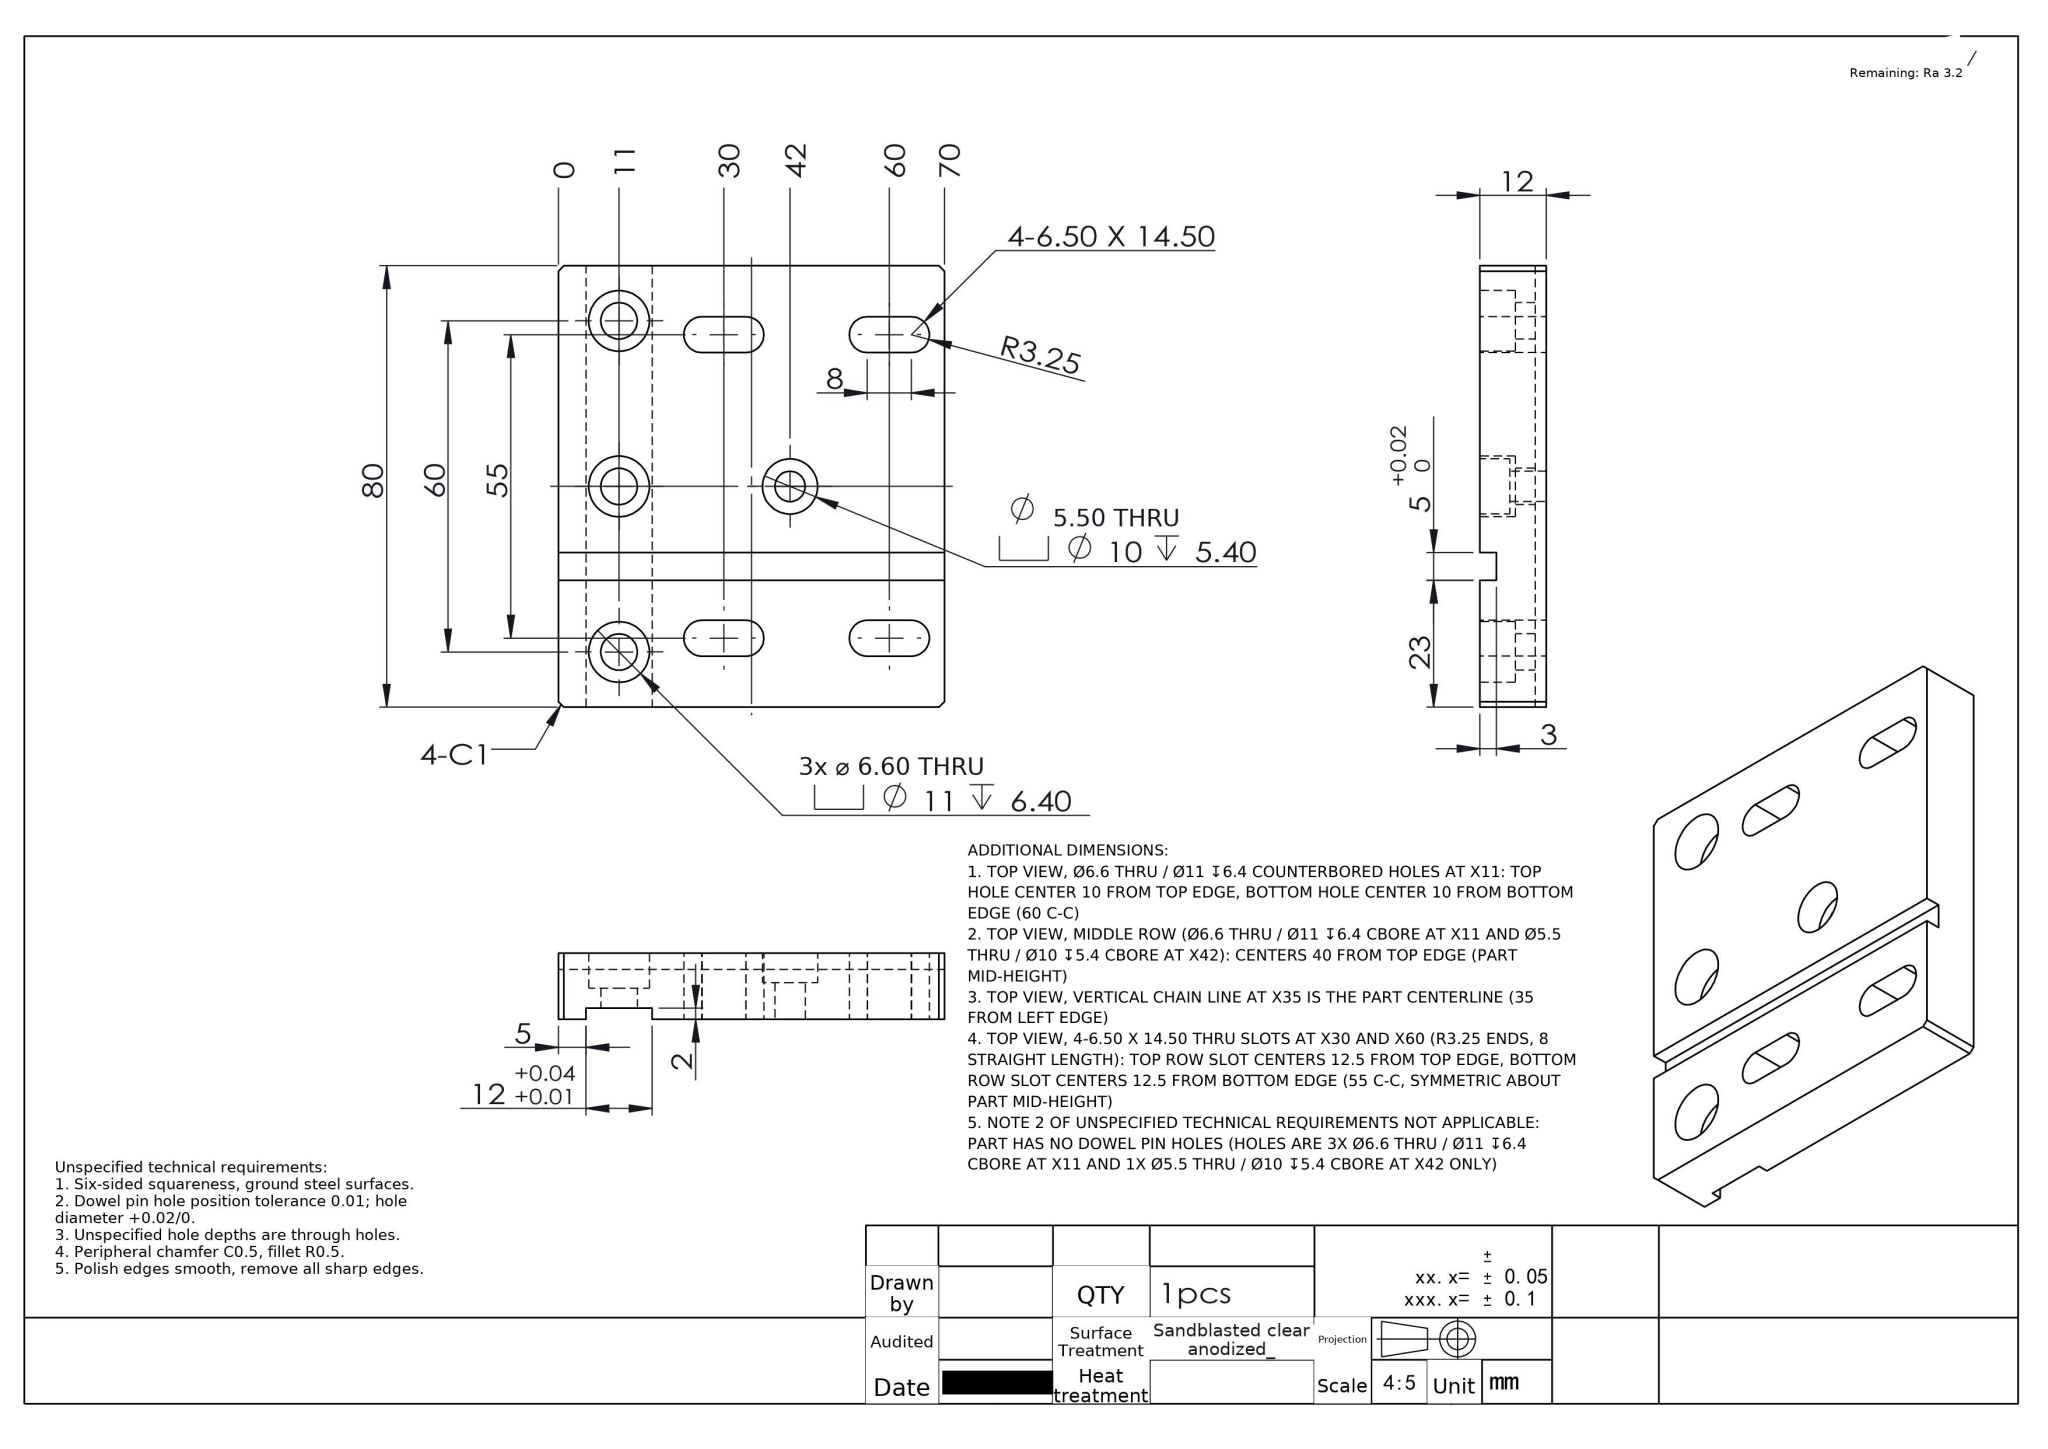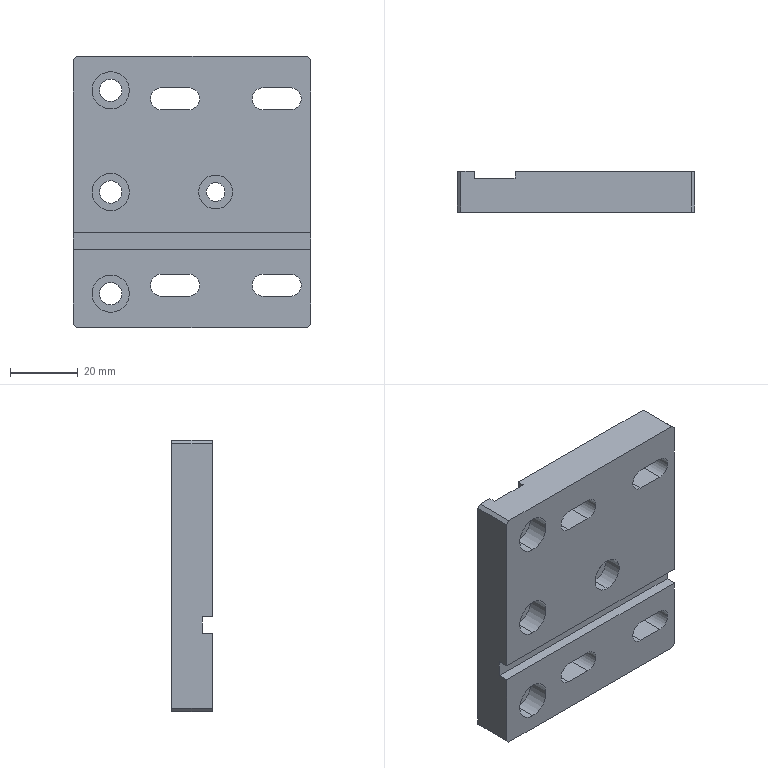Part | NX | mm | 1 solid | 54 faces | box 70 x 12 x 80 mm | volume 57342 mm3 | plane 30 | cylinder 24 | commonest cylinder face diameters 6.5 x8 11 x6 6.6 x6 10 x2 5.5 x2